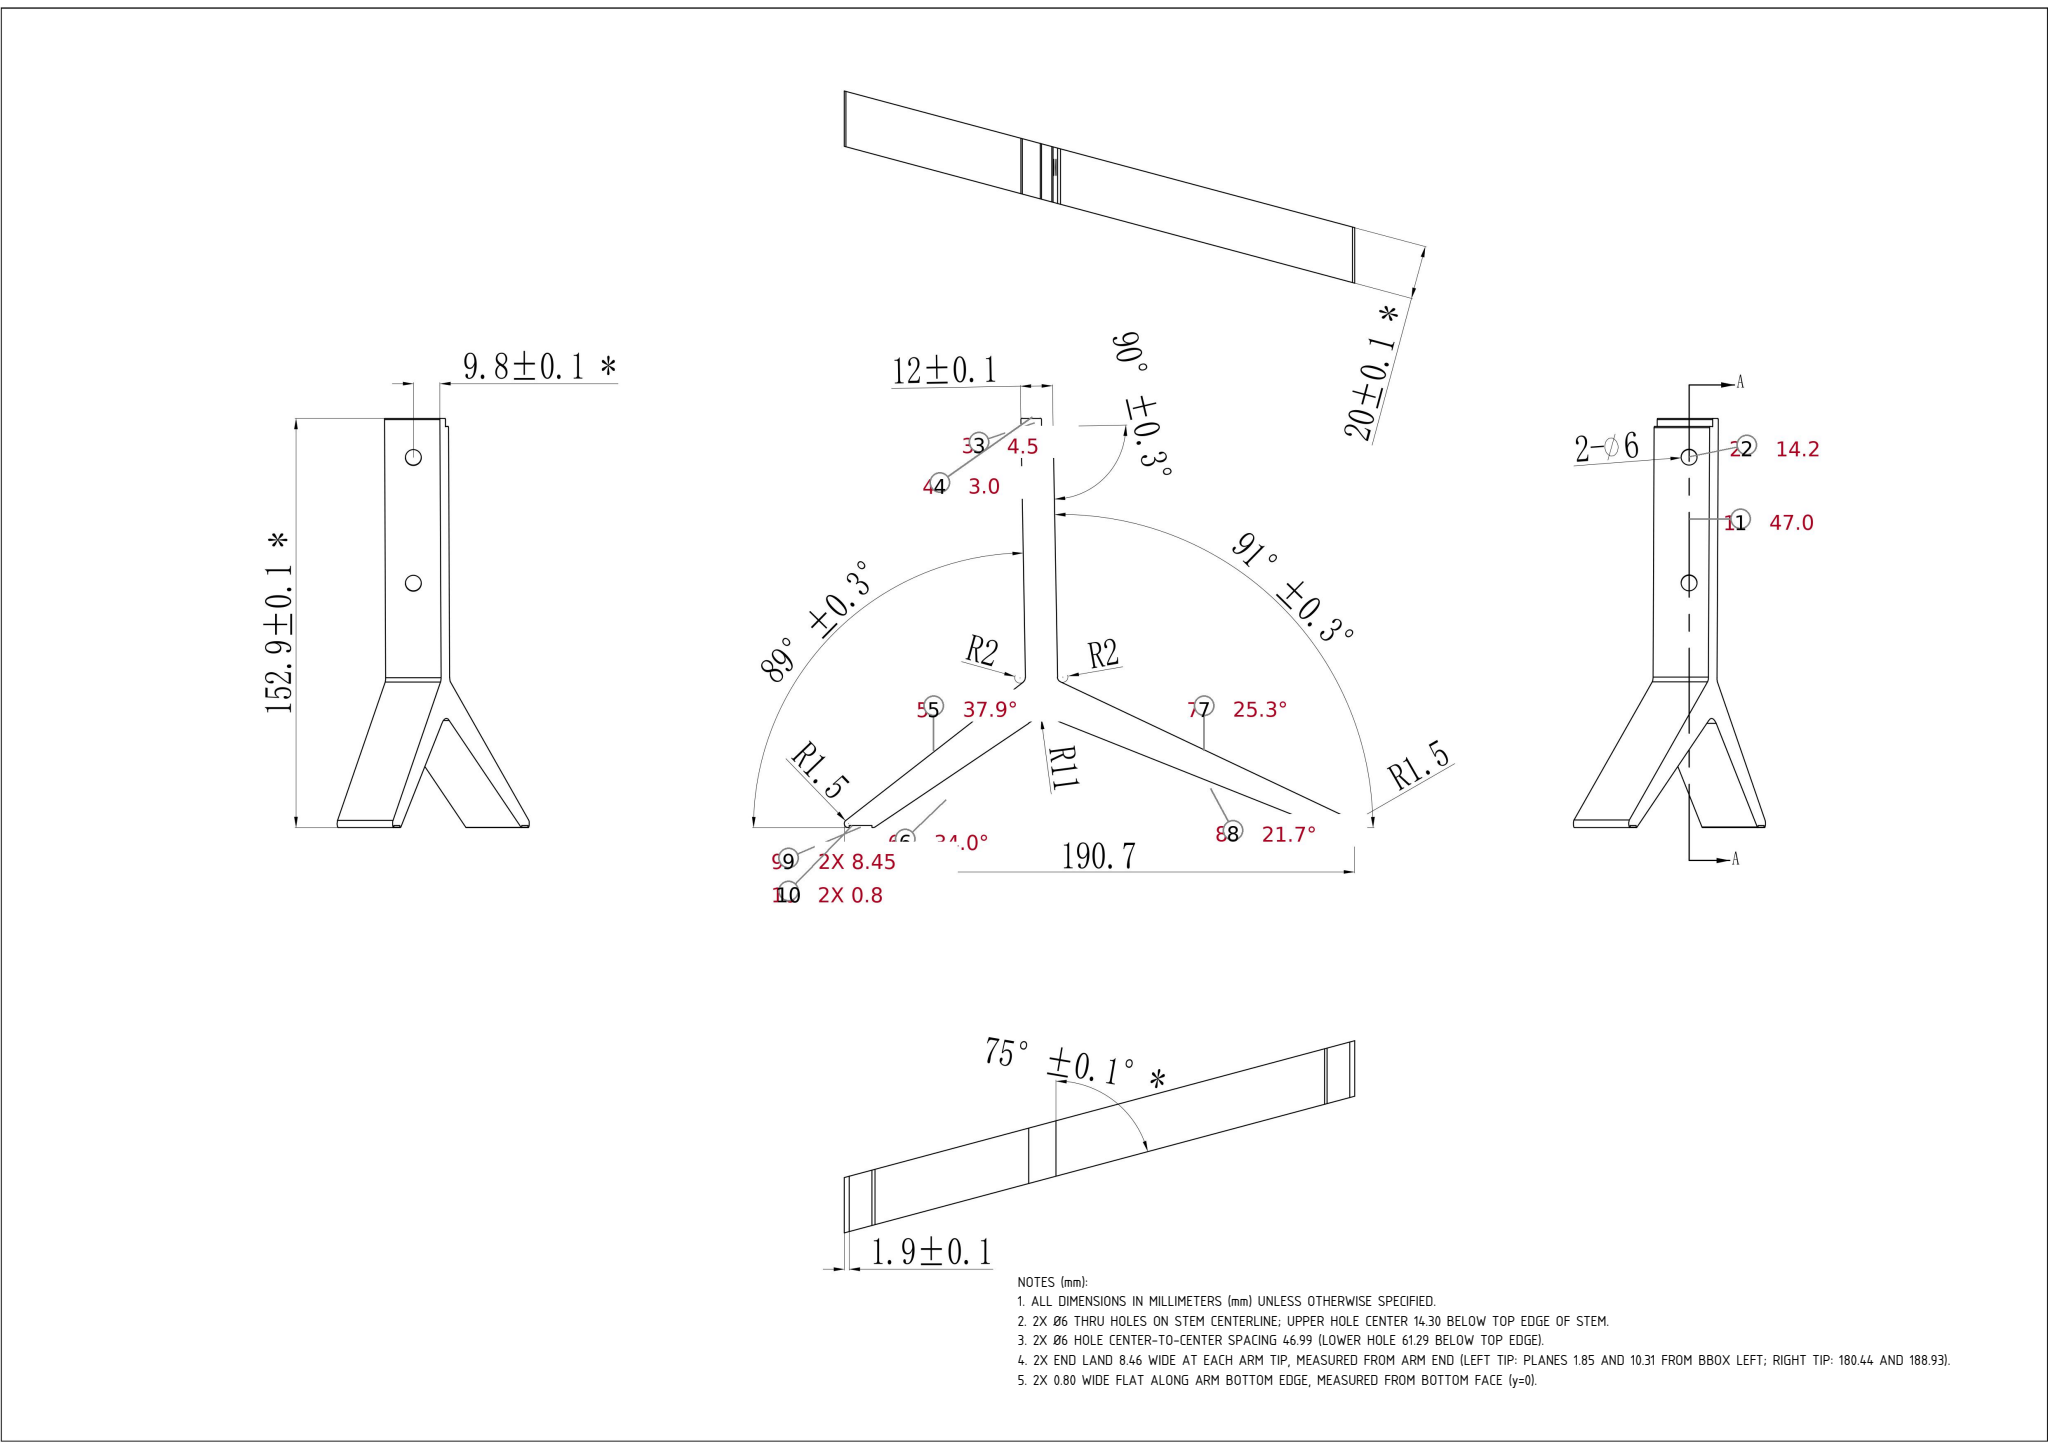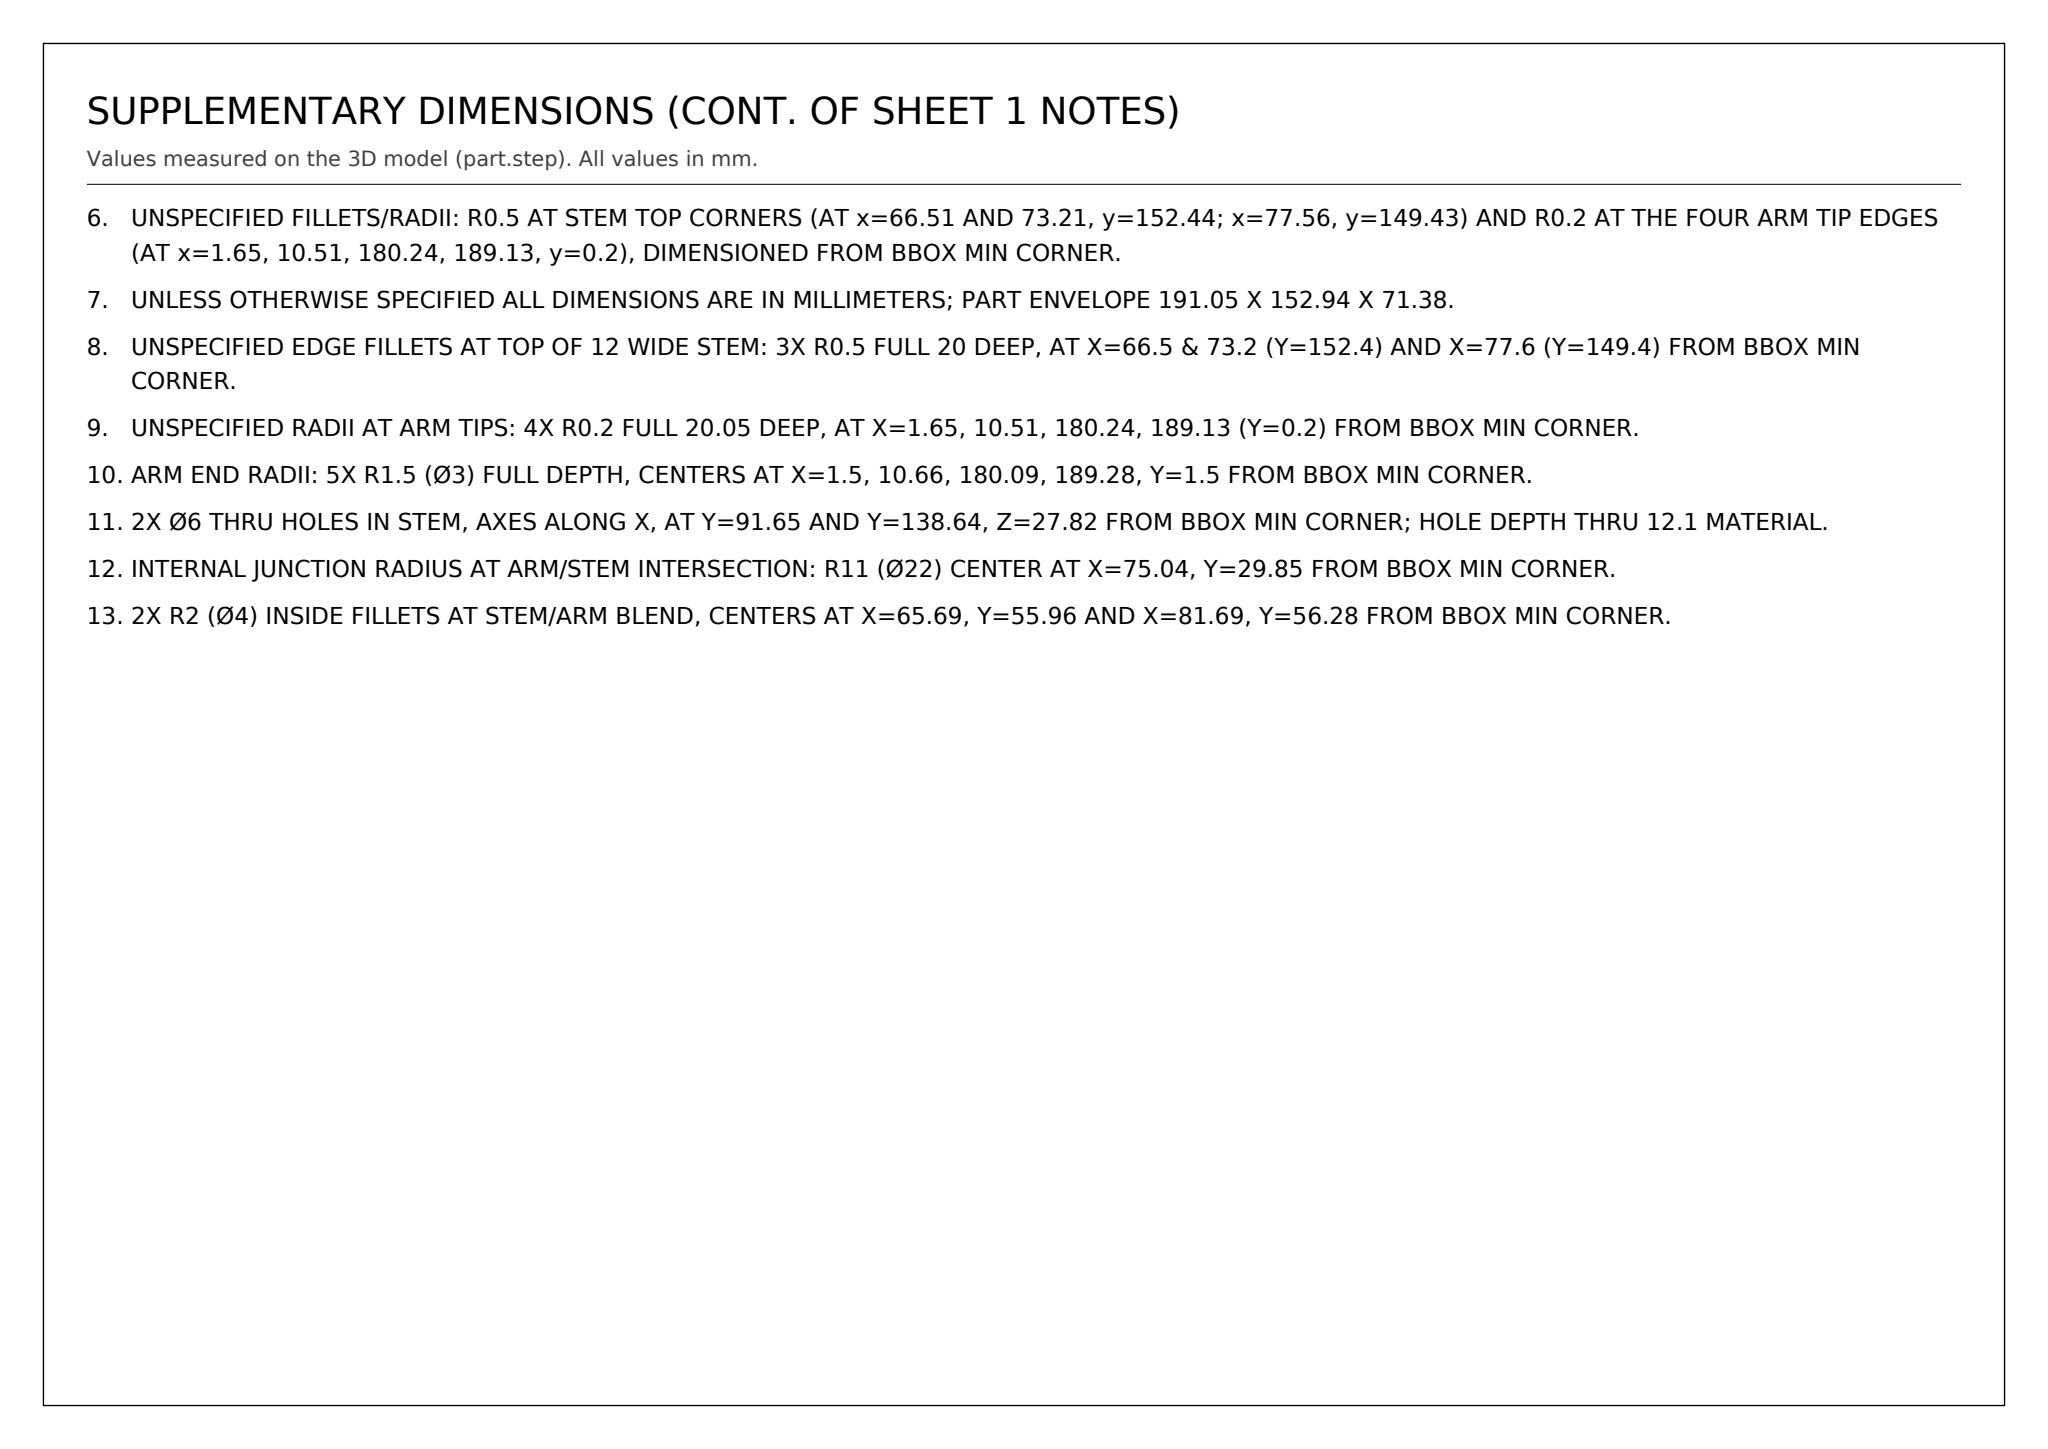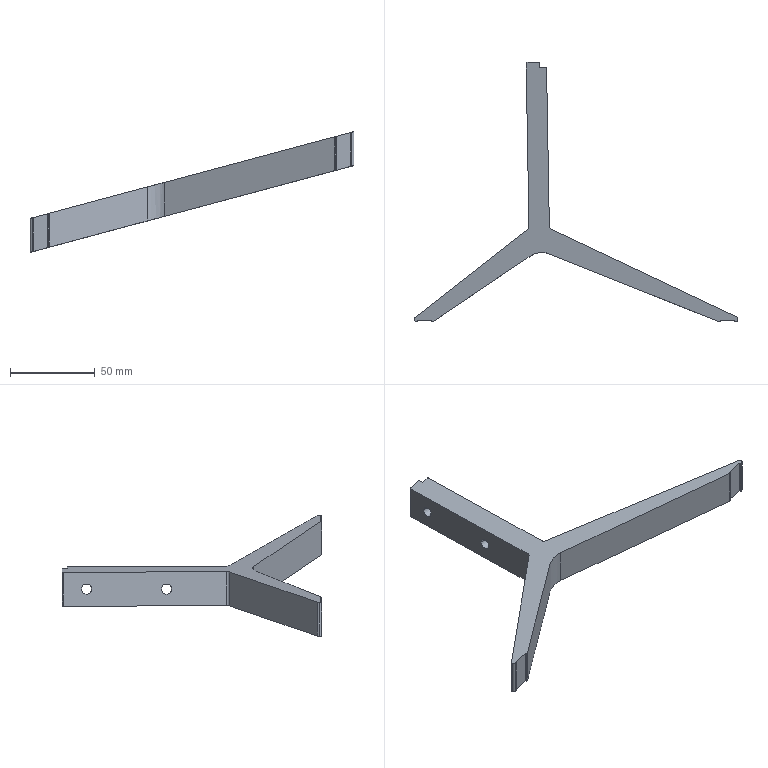Part | SolidWorks | mm | 1 solid | 41 faces | box 190.78 x 152.94 x 71.12 mm | volume 66917 mm3 | plane 21 | cylinder 20 | commonest cylinder face diameters 3 x5 6 x4 1 x4 0.4 x4 4 x2 22 x1
Drawing notes:
ALL DIMENSIONS IN MILLIMETERS (mm) UNLESS OTHERWISE SPECIFIED. | from the solid: STEP model units mm (bbox_xyz 191.053 x 152.94 x 71.382 mm)
2X Ø6 THRU HOLES ON STEM CENTERLINE; UPPER HOLE CENTER 14.30 BELOW TOP EDGE OF STEM. | from the solid: cylinders dia 6.0, axis x, pos y=138.64 (length 12.1) vs bbox y max 152.94 -> 14.30
2X Ø6 HOLE CENTER-TO-CENTER SPACING 46.99 (LOWER HOLE 61.29 BELOW TOP EDGE). | from the solid: cylinders dia 6.0, axis x, pos y=138.64 and y=91.65 -> 46.99 apart; 152.94-91.65=61.29
2X END LAND 8.46 WIDE AT EACH ARM TIP, MEASURED FROM ARM END (LEFT TIP: PLANES 1.85 AND 10.31 FROM BBOX LEFT; RIGHT TIP: 180.44 AND 188.93). | from the solid: axis_planes normal x at offsets 1.85, 10.31, 180.44, 188.93
2X 0.80 WIDE FLAT ALONG ARM BOTTOM EDGE, MEASURED FROM BOTTOM FACE (y=0). | from the solid: axis_planes normal y at offset 0.8 (count 2), bottom face y=0.0
UNSPECIFIED FILLETS/RADII: R0.5 AT STEM TOP CORNERS (AT x=66.51 AND 73.21, y=152.44; x=77.56, y=149.43) AND R0.2 AT THE FOUR ARM TIP EDGES (AT x=1.65, 10.51, 180.24, 189.13, y=0.2), DIMENSIONED FROM BBOX MIN CORNER. | from the solid: cylinders dia 1.0 at (66.51,152.44),(73.21,152.44),(77.56,149.43) = R0.5; cylinders dia 0.4 at (1.65,0.2),(10.51,0.2),(180.24,0.2),(189.13,0.2) = R0.2
UNLESS OTHERWISE SPECIFIED ALL DIMENSIONS ARE IN MILLIMETERS; PART ENVELOPE 191.05 X 152.94 X 71.38. | from the solid: bbox_xyz [191.053, 152.94, 71.382] (mm)
UNSPECIFIED EDGE FILLETS AT TOP OF 12 WIDE STEM: 3X R0.5 FULL 20 DEEP, AT X=66.5 & 73.2 (Y=152.4) AND X=77.6 (Y=149.4) FROM BBOX MIN CORNER. | from the solid: cylinders dia 1.0, axis z, pos (66.51,152.44), (73.21,152.44), (77.56,149.43), length ~20.1
UNSPECIFIED RADII AT ARM TIPS: 4X R0.2 FULL 20.05 DEEP, AT X=1.65, 10.51, 180.24, 189.13 (Y=0.2) FROM BBOX MIN CORNER. | from the solid: cylinders dia 0.4, axis z, pos (1.65,0.2), (10.51,0.2), (180.24,0.2), (189.13,0.2), length 20.05
ARM END RADII: 5X R1.5 (Ø3) FULL DEPTH, CENTERS AT X=1.5, 10.66, 180.09, 189.28, Y=1.5 FROM BBOX MIN CORNER. | from the solid: cylinders dia 3.0, axis z, pos (1.5,1.5), (10.66,1.5), (180.09,1.5), (189.28,1.5)
2X Ø6 THRU HOLES IN STEM, AXES ALONG X, AT Y=91.65 AND Y=138.64, Z=27.82 FROM BBOX MIN CORNER; HOLE DEPTH THRU 12.1 MATERIAL. | from the solid: cylinders dia 6.0, axis x, pos_other (y=91.65, z=27.82) and (y=138.64, z=27.82), length 12.1, count 2 each
INTERNAL JUNCTION RADIUS AT ARM/STEM INTERSECTION: R11 (Ø22) CENTER AT X=75.04, Y=29.85 FROM BBOX MIN CORNER. | from the solid: cylinder dia 22.0, axis z, pos (75.04, 29.85), length 22.74
2X R2 (Ø4) INSIDE FILLETS AT STEM/ARM BLEND, CENTERS AT X=65.69, Y=55.96 AND X=81.69, Y=56.28 FROM BBOX MIN CORNER. | from the solid: cylinders dia 4.0, axis z, pos (65.69,55.96) and (81.69,56.28)